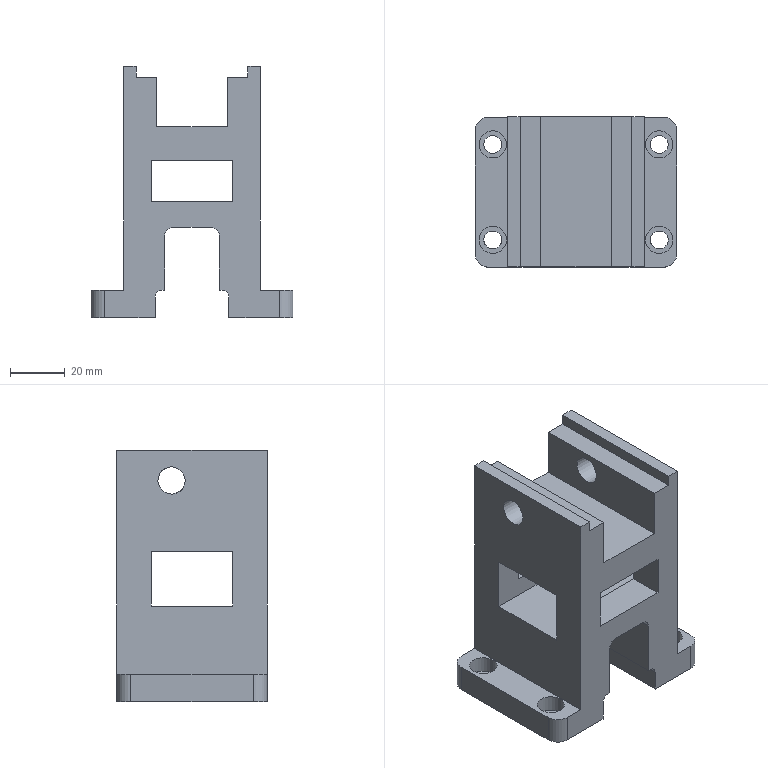Component | NX | WORK_TABLE | 1 solid | 58 faces | volume 143618 mm3 | plane 40 | cylinder 18 | commonest cylinder face diameters 10 x10 6.6 x4 5 x2 6 x2